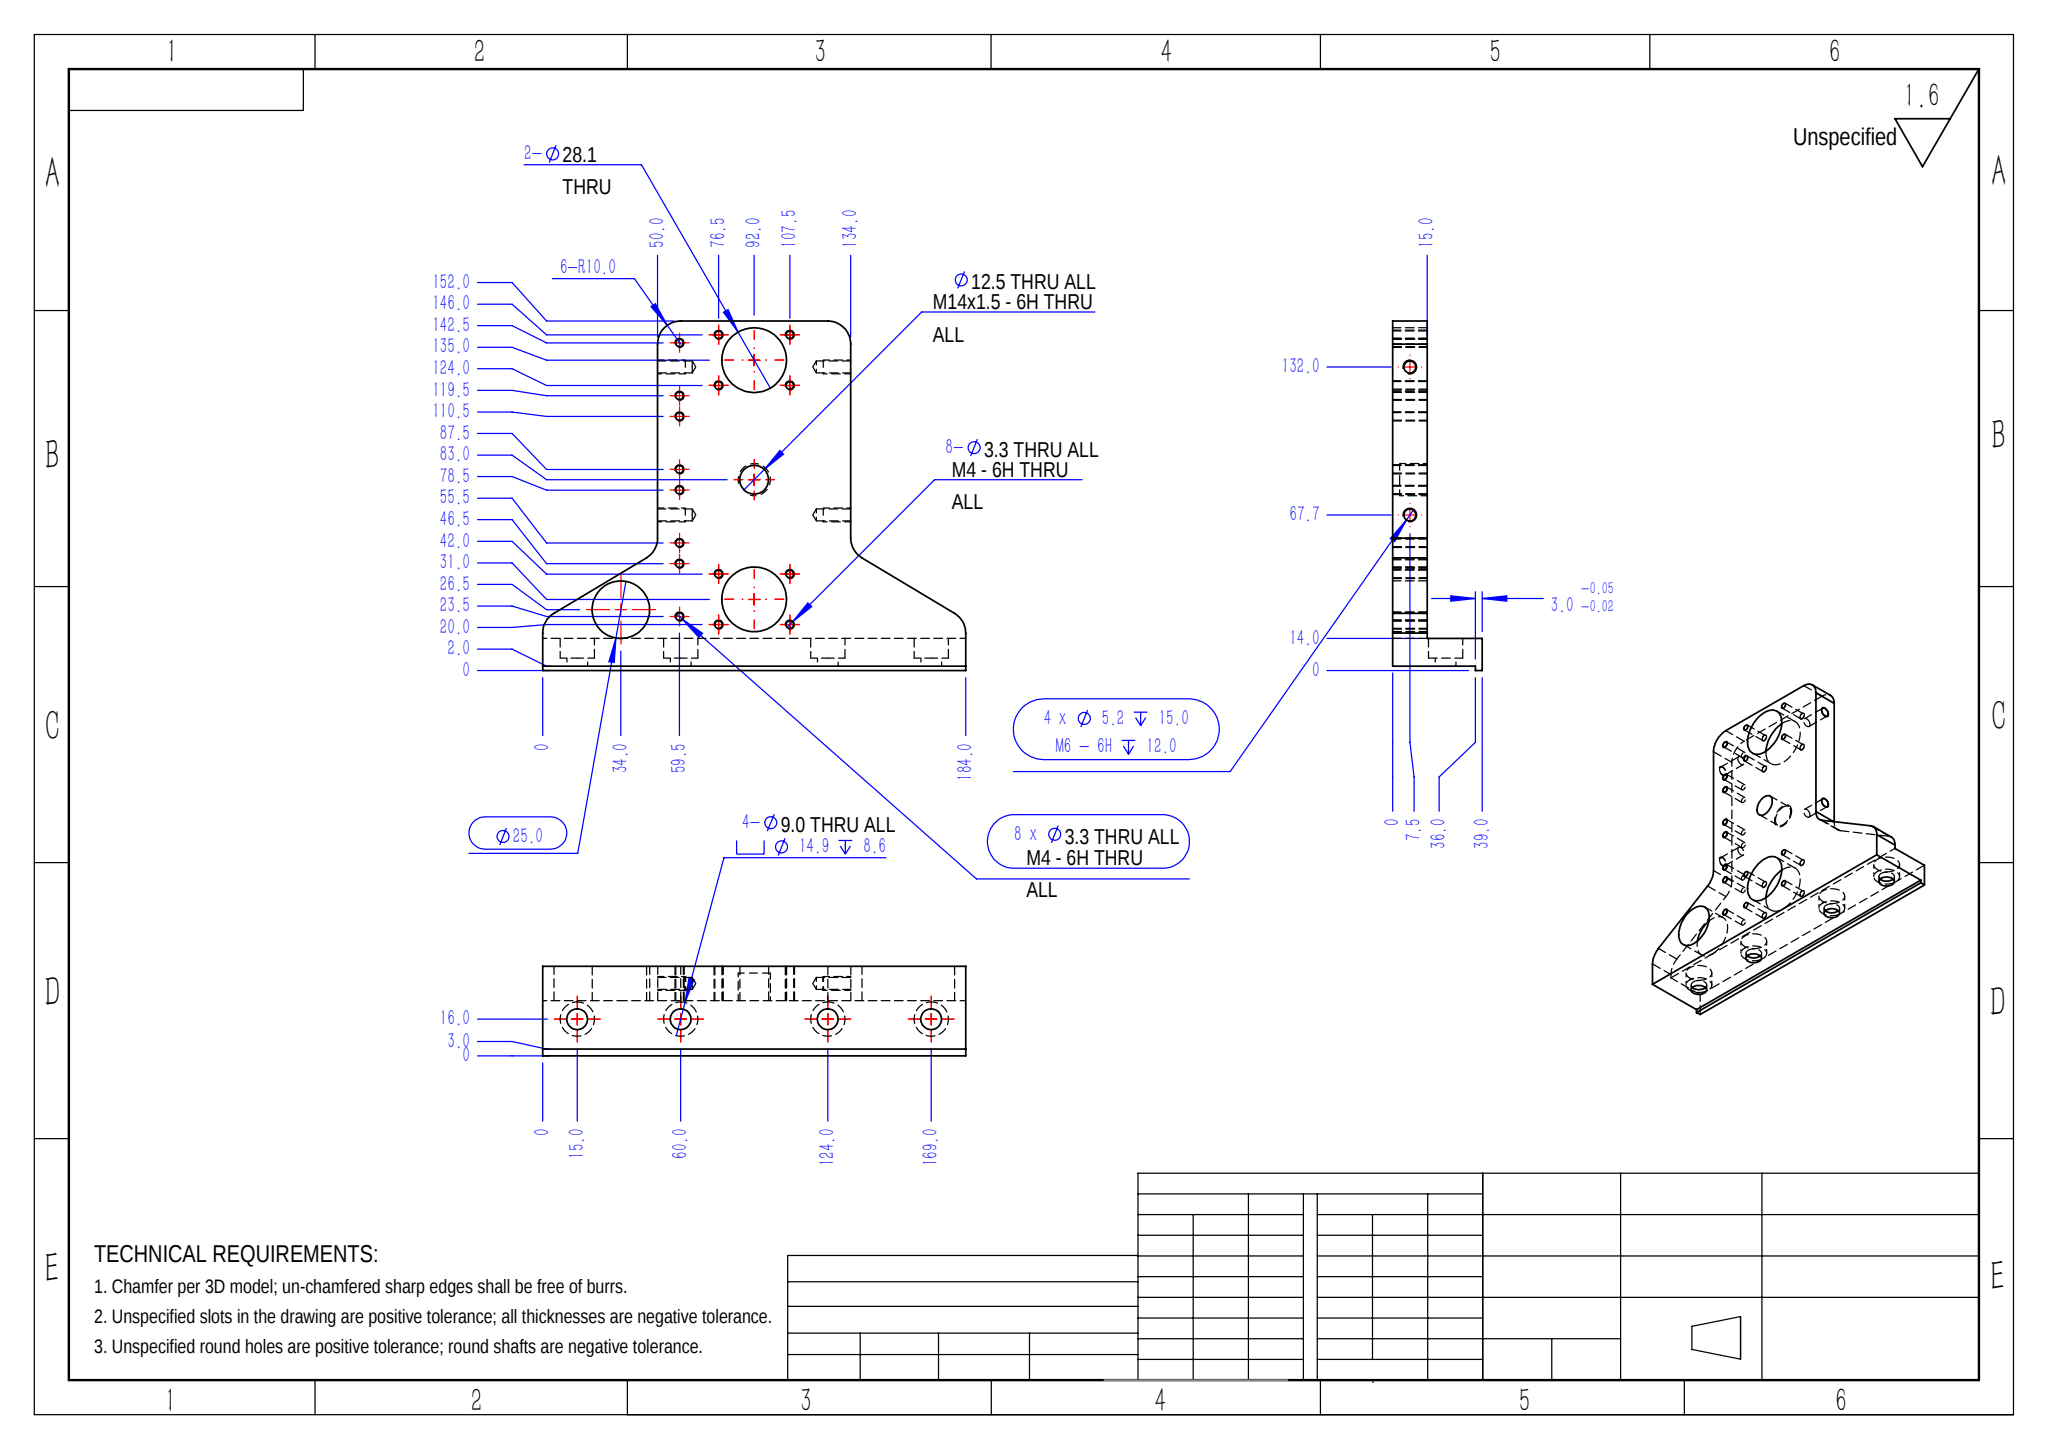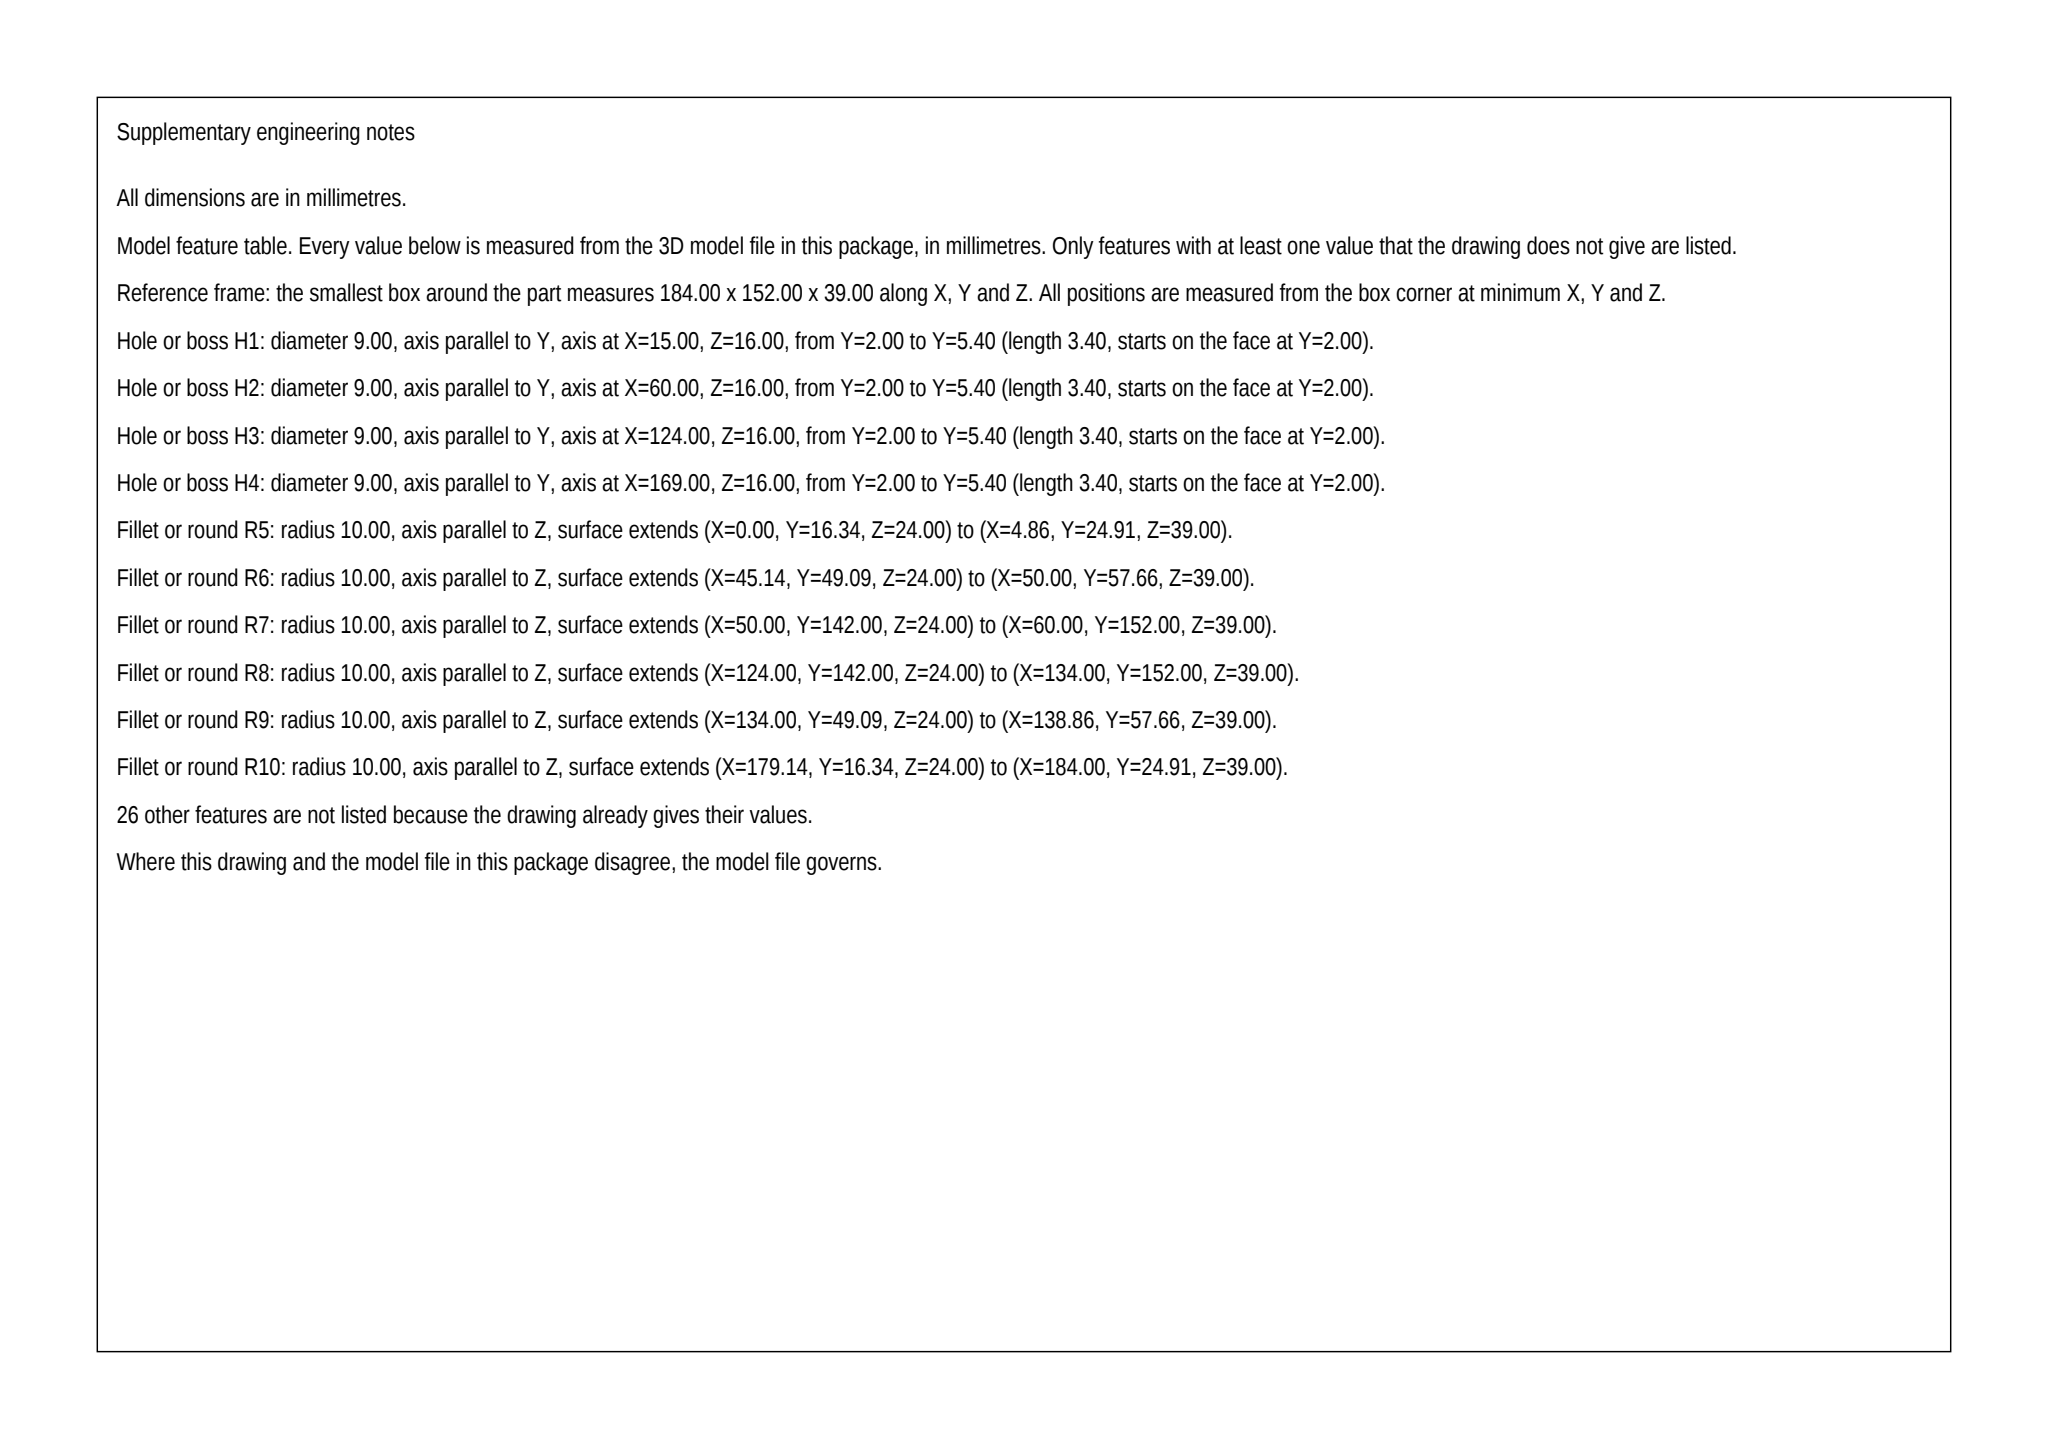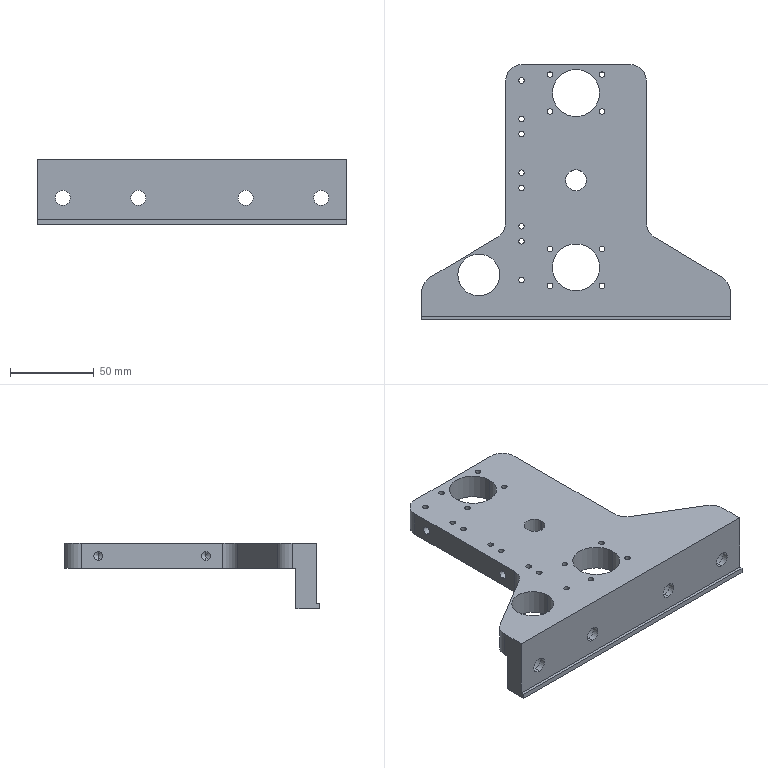Part | SolidWorks | mm | 1 solid | 96 faces | box 184 x 152 x 39 mm | volume 256909 mm3 | cylinder 70 | plane 18 | cone 8 | commonest cylinder face diameters 3.3 x32 5.2 x8 14.9 x8 9 x8 20 x6 28.1 x4 25 x2 12.5 x2
Drawing notes:
OVERALL 184.0 x 152.0 x 39.0 | from the solid: bbox_xyz [184.0,152.0,39.0]
GUSSET SLOPE 54° FROM BASE TOP Y14.0, BLEND R10.0 EA END | from the solid: R10 centers (10,16.34)&(40,57.66): dx=30, dy=41.32 -> 54.0 deg; base top plane y=14.0; 6 x Ø20 (R10.0) cyls
4X M6 SIDE HOLES AT Z31.5, Ø5.2 DP 15.0 FROM EA SIDE FACE X50/X134 | from the solid: cyl Ø5.2 axis x at [y=67.66,z=31.5] & [y=132.0,z=31.5], len 15.0, qty 4; planes x=50.0 and x=134.0
Ø25.0 THRU (15.0 THK PLATE) AT X34.0, Y26.5 | from the solid: cylinder [25.0,'z',[34.0,26.5],len 15.0]; z planes 24.0 to 39.0 = 15 thk
build123d program:
from build123d import *

# Parameters (mm, degrees)
SKETCH1_W                                       = 184
SKETCH1_H                                       = 150
BOSS_EXTRUDE1_DEPTH                             = 7.5
SKETCH2_W                                       = 184
SKETCH2_H                                       = 12
BOSS_EXTRUDE2_DEPTH                             = 24
CUT_EXTRUDE1_DEPTH                              = 64
FILLET1_R                                       = 10
FILLET2_R                                       = 10
FILLET3_R                                       = 10
SKETCH4_R                                       = 14.05
CUT_EXTRUDE2_DEPTH                              = 122.099
M14X1_5_TAPPED_HOLE1_D                          = 12.5
SKETCH7_W                                       = 184
SKETCH7_H                                       = 3
BOSS_EXTRUDE3_DEPTH                             = 2
M4_TAPPED_HOLE1_D                               = 3.3
M8_HEX_SOCKET_HEAD_CAP_SCREW_CBORE1_D           = 9
M8_HEX_SOCKET_HEAD_CAP_SCREW_CBORE1_CBORE_D     = 14.9
M8_HEX_SOCKET_HEAD_CAP_SCREW_CBORE1_CBORE_DEPTH = 8.6
M6_TAPPED_HOLE1_AT_2_COUNT                      = 2
M6_TAPPED_HOLE1_AT_2_PITCH                      = 64.338
M4_TAPPED_HOLE2_D                               = 3.3
LPATTERN1_COUNT                                 = 4
LPATTERN1_PITCH                                 = 32
SKETCH16_R                                      = 12.5
CUT_EXTRUDE3_DEPTH                              = 42


with BuildPart() as part:
    # Sketch1 → Boss-Extrude1 (new, symmetric)
    with BuildSketch(Plane.XY):
        Rectangle(SKETCH1_W, SKETCH1_H)
    extrude(amount=BOSS_EXTRUDE1_DEPTH, both=True)

    # Sketch2 → Boss-Extrude2 (add)
    with BuildSketch(Plane(origin=(0, 0, -7.5), x_dir=(-1, 0, 0), z_dir=(0, 0, -1))):
        with Locations((0, -69)):
            Rectangle(SKETCH2_W, SKETCH2_H)
    extrude(amount=BOSS_EXTRUDE2_DEPTH)

    # Sketch3 → Cut-Extrude1 (cut)
    with BuildSketch(Plane(origin=(0, 0, -7.5), x_dir=(-1, 0, 0), z_dir=(0, 0, -1))):
        Polygon((92, -55), (42, -25), (42, 75), (92, 75), align=None)
    cut_extrude1 = extrude(amount=-CUT_EXTRUDE1_DEPTH, mode=Mode.SUBTRACT)

    # Mirror1: Cut-Extrude1 across plane
    add(cut_extrude1.mirror(Plane(origin=(0, 0, 0), x_dir=(0, 0, 1), z_dir=(1, 0, 0))), mode=Mode.SUBTRACT)

    # Fillet1
    fillet1_edges = [part.edges().sort_by_distance(p)[0] for p in [
        (-42, 75, 0),
        (42, 75, 0),
    ]]
    fillet(fillet1_edges, radius=FILLET1_R)

    # Fillet2
    fillet2_edges = [part.edges().sort_by_distance(p)[0] for p in [
        (-42, -25, 0),
        (42, -25, 0),
    ]]
    fillet(fillet2_edges, radius=FILLET2_R)

    # Fillet3
    fillet3_edges = [part.edges().sort_by_distance(p)[0] for p in [
        (-92, -55, 0),
        (92, -55, 0),
    ]]
    fillet(fillet3_edges, radius=FILLET3_R)

    # Sketch4 → Cut-Extrude2 (cut, through all)
    with BuildSketch(Plane(origin=(0, 0, -7.5), x_dir=(-1, 0, 0), z_dir=(0, 0, -1))):
        with Locations((0, 58)):
            Circle(SKETCH4_R)
    cut_extrude2 = extrude(amount=-CUT_EXTRUDE2_DEPTH, mode=Mode.SUBTRACT)

    # Mirror2: Cut-Extrude2 across plane
    add(cut_extrude2.mirror(Plane.ZX.offset(6)), mode=Mode.SUBTRACT)

    # M14x1.5 Tapped Hole1 (through all)
    with Locations(Plane(origin=(0, 0, -7.5), x_dir=(-1, 0, 0), z_dir=(0, 0, -1))):
        with Locations((0, 6)):
            Hole(M14X1_5_TAPPED_HOLE1_D / 2)

    # Sketch7 → Boss-Extrude3 (add)
    with BuildSketch(Plane.XZ.offset(75)):
        with Locations((0, -30)):
            Rectangle(SKETCH7_W, SKETCH7_H)
    extrude(amount=BOSS_EXTRUDE3_DEPTH)

    # M4 Tapped Hole1 (through all)
    with Locations(Plane(origin=(0, 0, -7.5), x_dir=(-1, 0, 0), z_dir=(0, 0, -1))):
        with Locations((15.5, 69), (-15.5, 69), (15.5, 47), (-15.5, 47), (15.5, -35), (-15.5, -35), (15.5, -57), (-15.5, -57)):
            Hole(M4_TAPPED_HOLE1_D / 2)

    # M8 Hex Socket Head Cap Screw CBORE1 (through all)
    with Locations(Plane(origin=(0, -63, 0), x_dir=(1, 0, 0), z_dir=(0, 1, 0))):
        with Locations((-77, 15.5), (-32, 15.5)):
            m8_hex_socket_head_cap_screw_cbore1 = CounterBoreHole(M8_HEX_SOCKET_HEAD_CAP_SCREW_CBORE1_D / 2, M8_HEX_SOCKET_HEAD_CAP_SCREW_CBORE1_CBORE_D / 2, M8_HEX_SOCKET_HEAD_CAP_SCREW_CBORE1_CBORE_DEPTH)

    # Mirror3: M8 Hex Socket Head Cap Screw CBORE1 across plane
    add(m8_hex_socket_head_cap_screw_cbore1.mirror(Plane(origin=(0, 0, 0), x_dir=(0, 0, 1), z_dir=(1, 0, 0))), mode=Mode.SUBTRACT)

    # Sketch13 → M6 Tapped Hole1 (revolve, cut)
    with BuildSketch(Plane(origin=(42, 55, 0), x_dir=(0, 0, -1), z_dir=(0, 1, 0))):
        Polygon((0, 0), (0, 16.562), (2.6, 15), (2.6, 0), align=None)
    m6_tapped_hole1 = revolve(axis=Axis((48.35, 55, 0), (-1, 0, 0)), mode=Mode.SUBTRACT)

    # M6 Tapped Hole1 at 2: M6 Tapped Hole1 ×2
    with Locations(*[(0, -i * M6_TAPPED_HOLE1_AT_2_PITCH, 0) for i in range(1, M6_TAPPED_HOLE1_AT_2_COUNT)]):
        add(m6_tapped_hole1, mode=Mode.SUBTRACT)

    # Mirror4: M6 Tapped Hole1 across plane
    add(m6_tapped_hole1.mirror(Plane(origin=(0, 0, 0), x_dir=(0, 0, 1), z_dir=(1, 0, 0))), mode=Mode.SUBTRACT)

    # Mirror4 copy 1 sketch → Mirror4 copy 1 (revolve, cut)
    with BuildSketch(Plane(origin=(-42, -9.338, 0), x_dir=(0, 0, -1), z_dir=(0, 1, 0))):
        Polygon((0, 0), (0, -16.562), (2.6, -15), (2.6, 0), align=None)
    revolve(axis=Axis((-48.35, -9.338, 0), (-1, 0, 0)), mode=Mode.SUBTRACT)

    # M4 Tapped Hole2 (through all)
    with Locations(Plane.XY.offset(7.5)):
        with Locations((-32.5, 65.5), (-32.5, 42.5)):
            m4_tapped_hole2 = Hole(M4_TAPPED_HOLE2_D / 2)

    # LPattern1: M4 Tapped Hole2 ×4
    with Locations(*[(0, -i * LPATTERN1_PITCH, 0) for i in range(1, LPATTERN1_COUNT)]):
        add(m4_tapped_hole2, mode=Mode.SUBTRACT)

    # Sketch16 → Cut-Extrude3 (cut)
    with BuildSketch(Plane(origin=(0, 0, -7.5), x_dir=(-1, 0, 0), z_dir=(0, 0, -1))):
        with Locations((58, -50.5)):
            Circle(SKETCH16_R)
    extrude(amount=-CUT_EXTRUDE3_DEPTH, mode=Mode.SUBTRACT)


solid = part.part